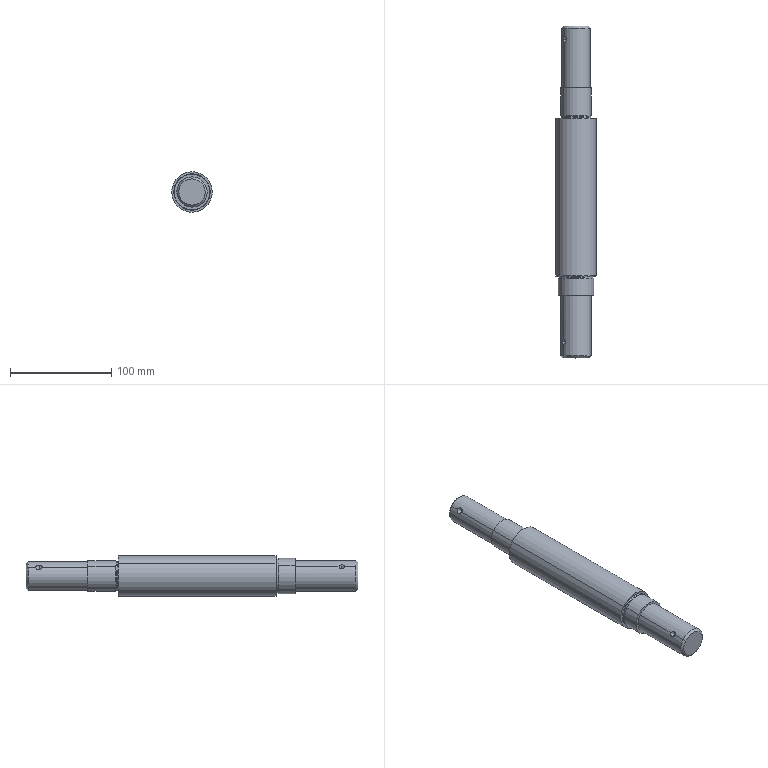Component | SolidWorks | 13-1 | 1 solid | 50 faces | volume 315340 mm3 | cylinder 22 | cone 12 | plane 12 | torus 4 | commonest cylinder face diameters 5 x8 30 x4 29 x2 40 x2 34.4 x2 35 x2 28 x2